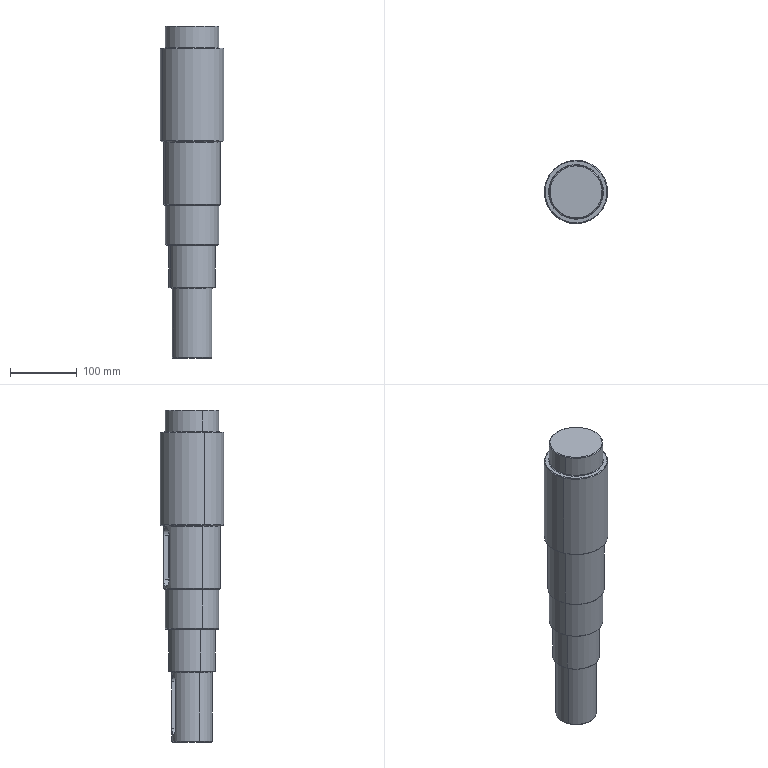Component | SolidWorks | PartAssemblyInLowerHousing-1_LowSpeedAxisAssembly-1_LowSpeedAxis-1 | 1 solid | 53 faces | box 95 x 95 x 497 mm | volume 2516140 mm3 | cylinder 16 | cone 14 | plane 13 | torus 10 | commonest cylinder face diameters 80 x4 95 x2 85 x2 70 x2 60 x2 22 x2 18 x2
build123d program:
from build123d import *

# Parameters (mm, degrees)
CUT_EXTRUDE2_DEPTH = 9
CUT_EXTRUDE3_DEPTH = 7
CHAMFER1_SIZE      = 1
FILLET1_R          = 1


with BuildPart() as part:
    # Sketch1 → Revolve2 (revolve)
    with BuildSketch(Plane.XY, mode=Mode.PRIVATE) as revolve2_sk:
        Polygon((0, 0), (0, 30), (105, 30), (105, 35), (169, 35), (169, 40), (229, 40), (229, 42.5), (324, 42.5), (324, 47.5), (464, 47.5), (464, 40), (497, 40), (497, 0), align=None)
    revolve(revolve2_sk.sketch.rotate(Axis((-10.324, 0, 0), (1, 0, 0)), 90), axis=Axis((-10.324, 0, 0), (1, 0, 0)))

    # Sketch2 → Cut-Extrude2 (cut)
    with BuildSketch(Plane(origin=(0, 42.5, 0), x_dir=(1, 0, 0), z_dir=(0, 1, 0))):
        with BuildLine():
            Line((309, 11), (244, 11))
            ThreePointArc((244, 11), (233, 0), (244, -11))
            Line((244, -11), (309, -11))
            ThreePointArc((309, -11), (320, 0), (309, 11))
        make_face()
    extrude(amount=-CUT_EXTRUDE2_DEPTH, mode=Mode.SUBTRACT)

    # Sketch4 → Cut-Extrude3 (cut)
    with BuildSketch(Plane(origin=(0, 30, 0), x_dir=(1, 0, 0), z_dir=(0, 1, 0))):
        with BuildLine():
            Line((90, 10.905), (20, 10.905))
            ThreePointArc((20, 10.905), (11, 1.905), (20, -7.095))
            Line((20, -7.095), (90, -7.095))
            ThreePointArc((90, -7.095), (99, 1.905), (90, 10.905))
        make_face()
    extrude(amount=-CUT_EXTRUDE3_DEPTH, mode=Mode.SUBTRACT)

    # Chamfer1
    chamfer1_edges = [part.edges().sort_by_distance(p)[0] for p in [
        (497, 0, -40),
        (464, 0, -47.5),
        (324, 0, -47.5),
        (229, 0, -42.5),
        (169, 0, -40),
        (105, 0, -35),
        (0, 0, -30),
    ]]
    chamfer(chamfer1_edges, length=CHAMFER1_SIZE)

    # Fillet1
    fillet1_edges = [part.edges().sort_by_distance(p)[0] for p in [
        (464, 0, -40),
        (324, 0, -42.5),
        (229, 0, -40),
        (169, 0, -35),
        (105, 0, -30),
    ]]
    fillet(fillet1_edges, radius=FILLET1_R)


solid = part.part

# Placed as in the assembly
solid = solid.moved(Location((1140.83, 1268.591, 1315.214), (90, -67.477, 90)))